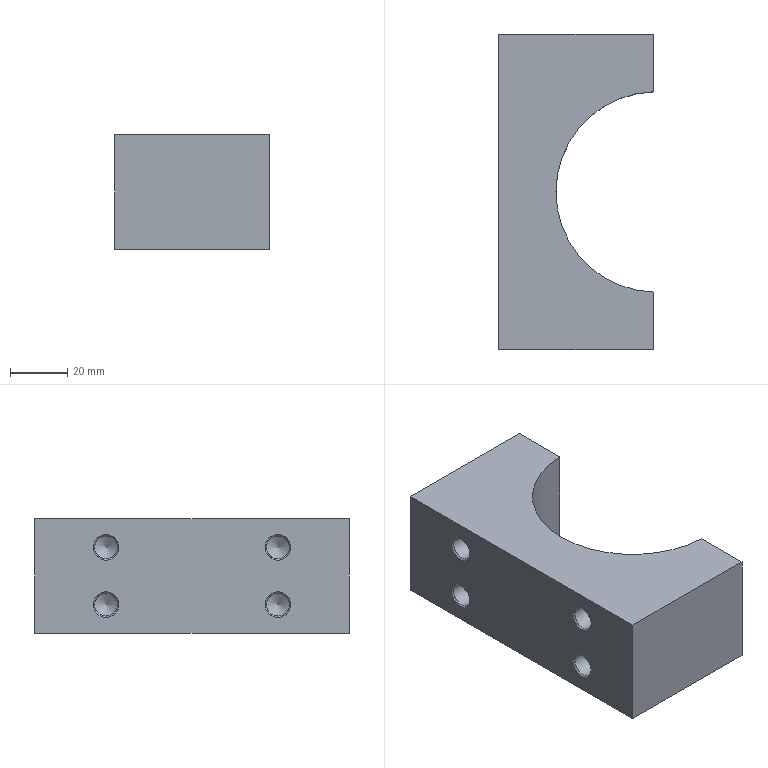Component | NX | CH3404_2-1 | 1 solid | 26 faces | volume 151530 mm3 | cone 12 | plane 7 | cylinder 7 | commonest cylinder face diameters 8 x4 10 x2 70 x1